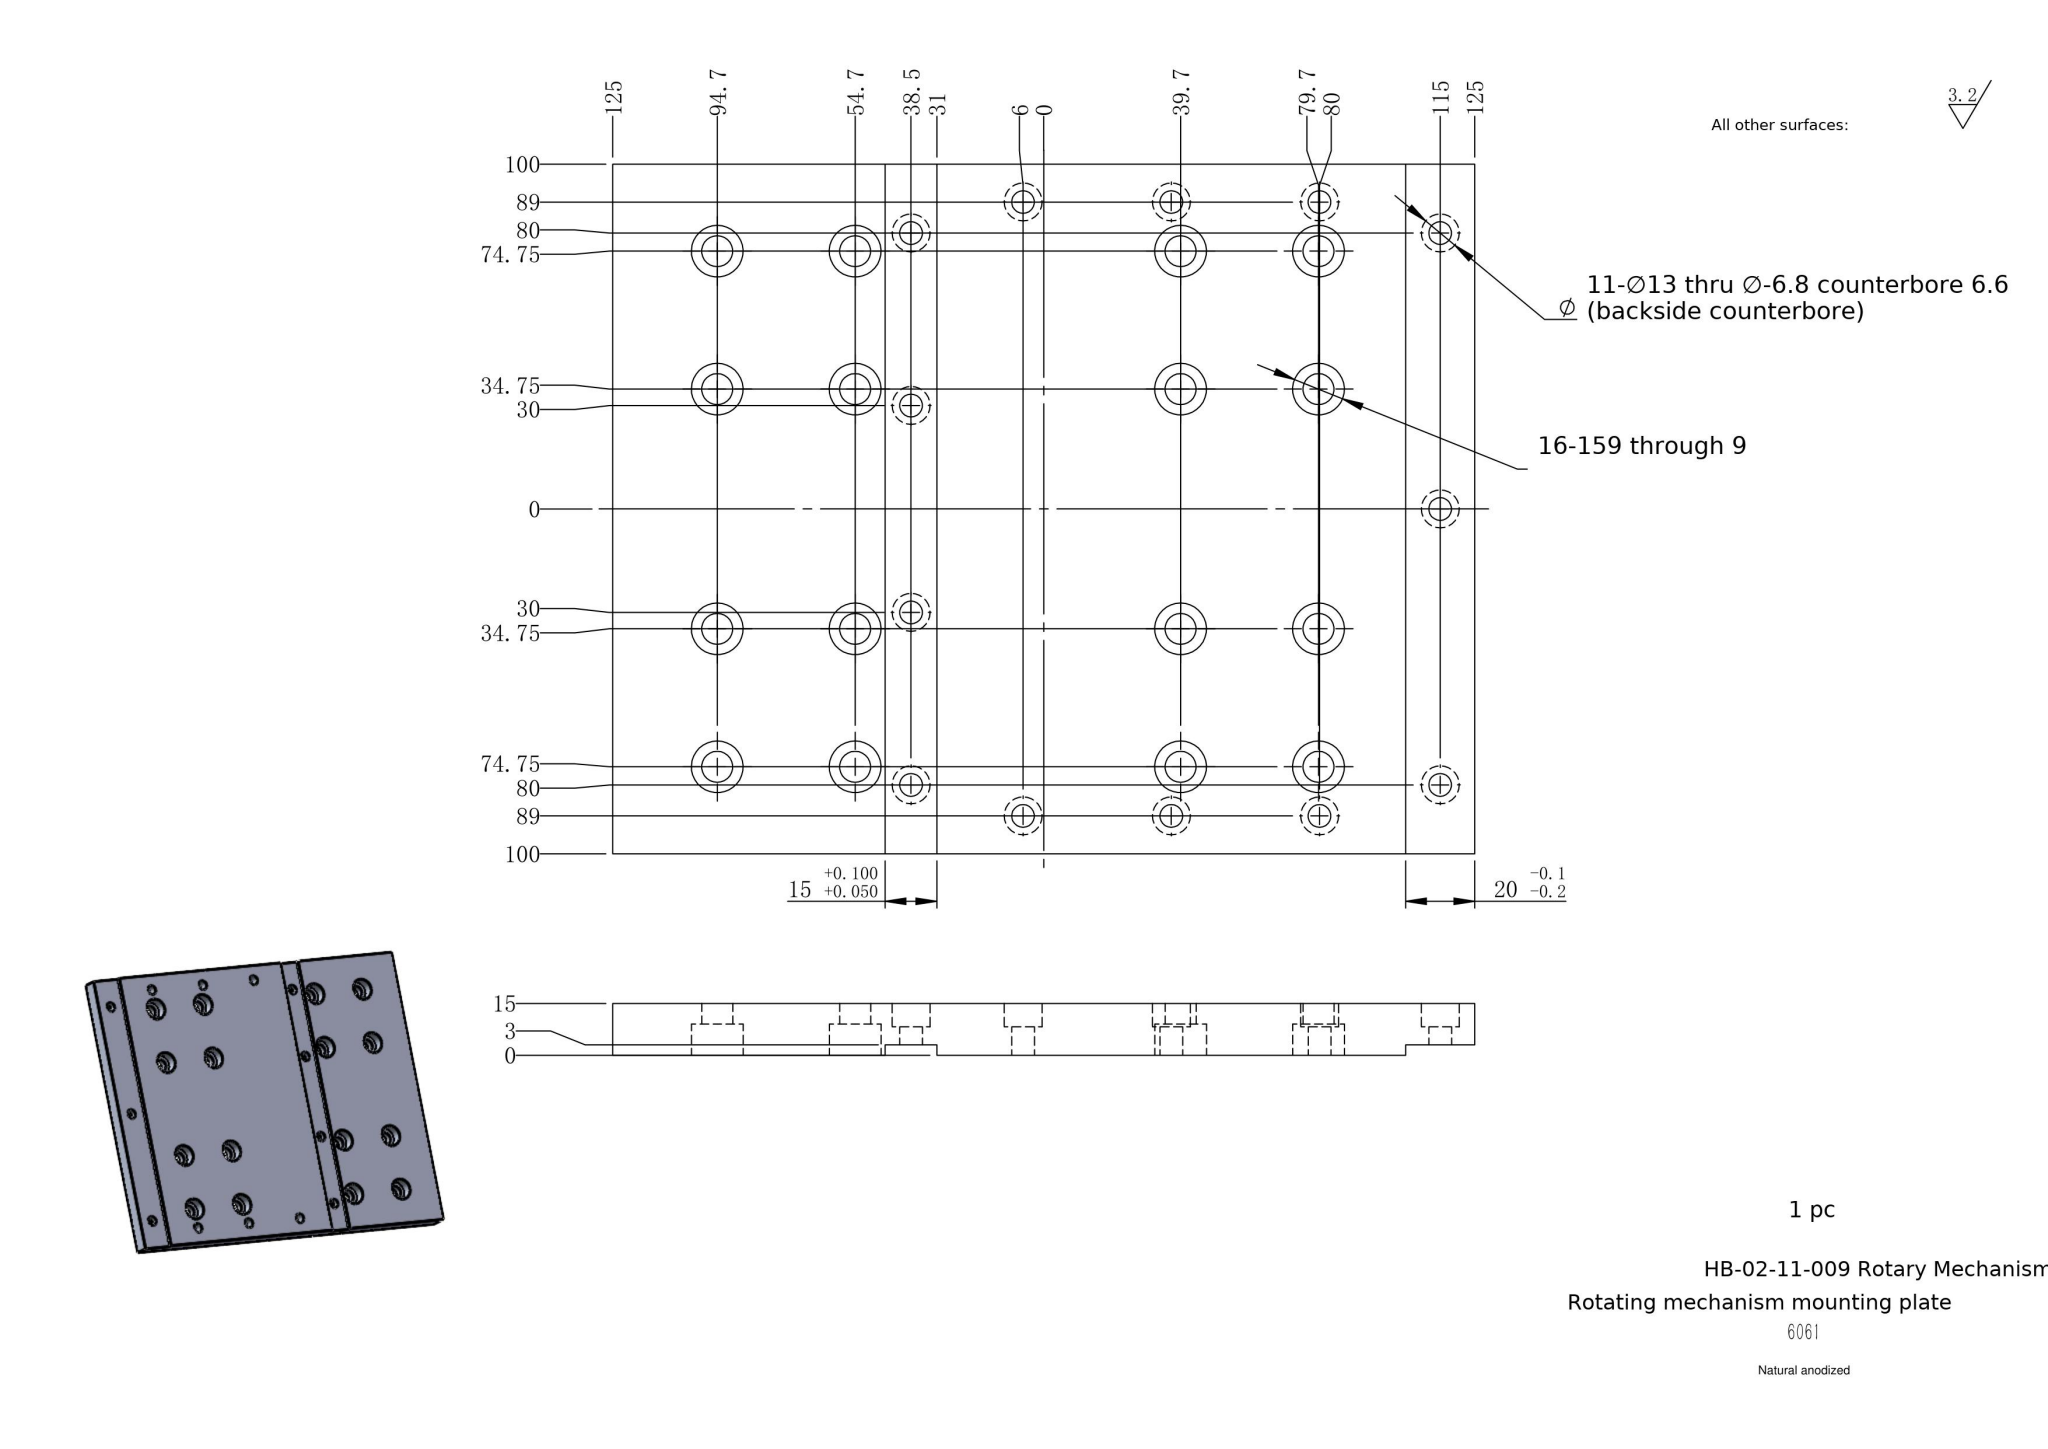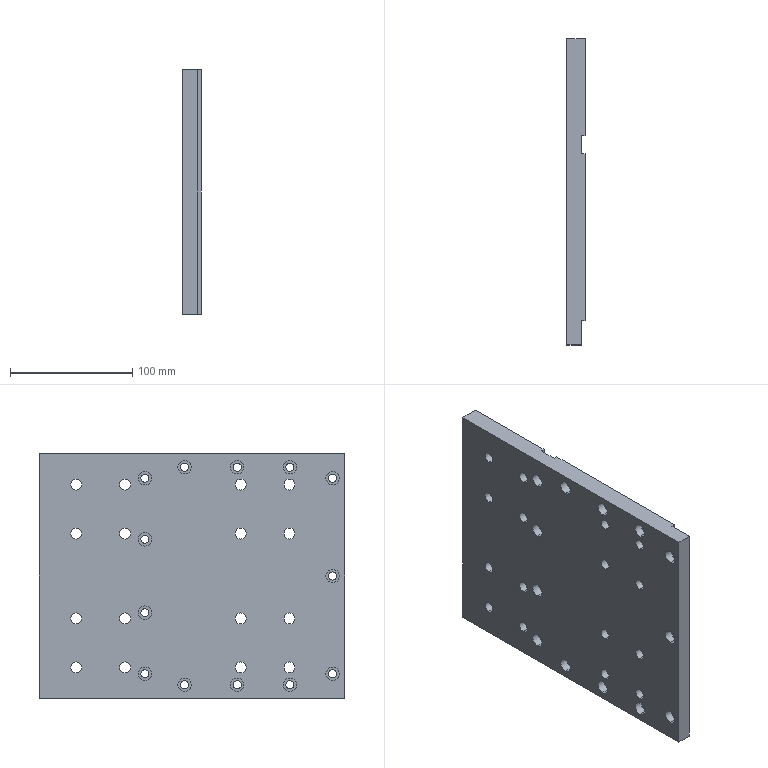Part | SolidWorks | mm | material 6061 | 1 solid | 157 faces | box 15 x 250 x 200 mm | volume 686116 mm3 | cylinder 116 | plane 41 | commonest cylinder face diameters 15 x32 9 x32 11 x26 6.6 x26